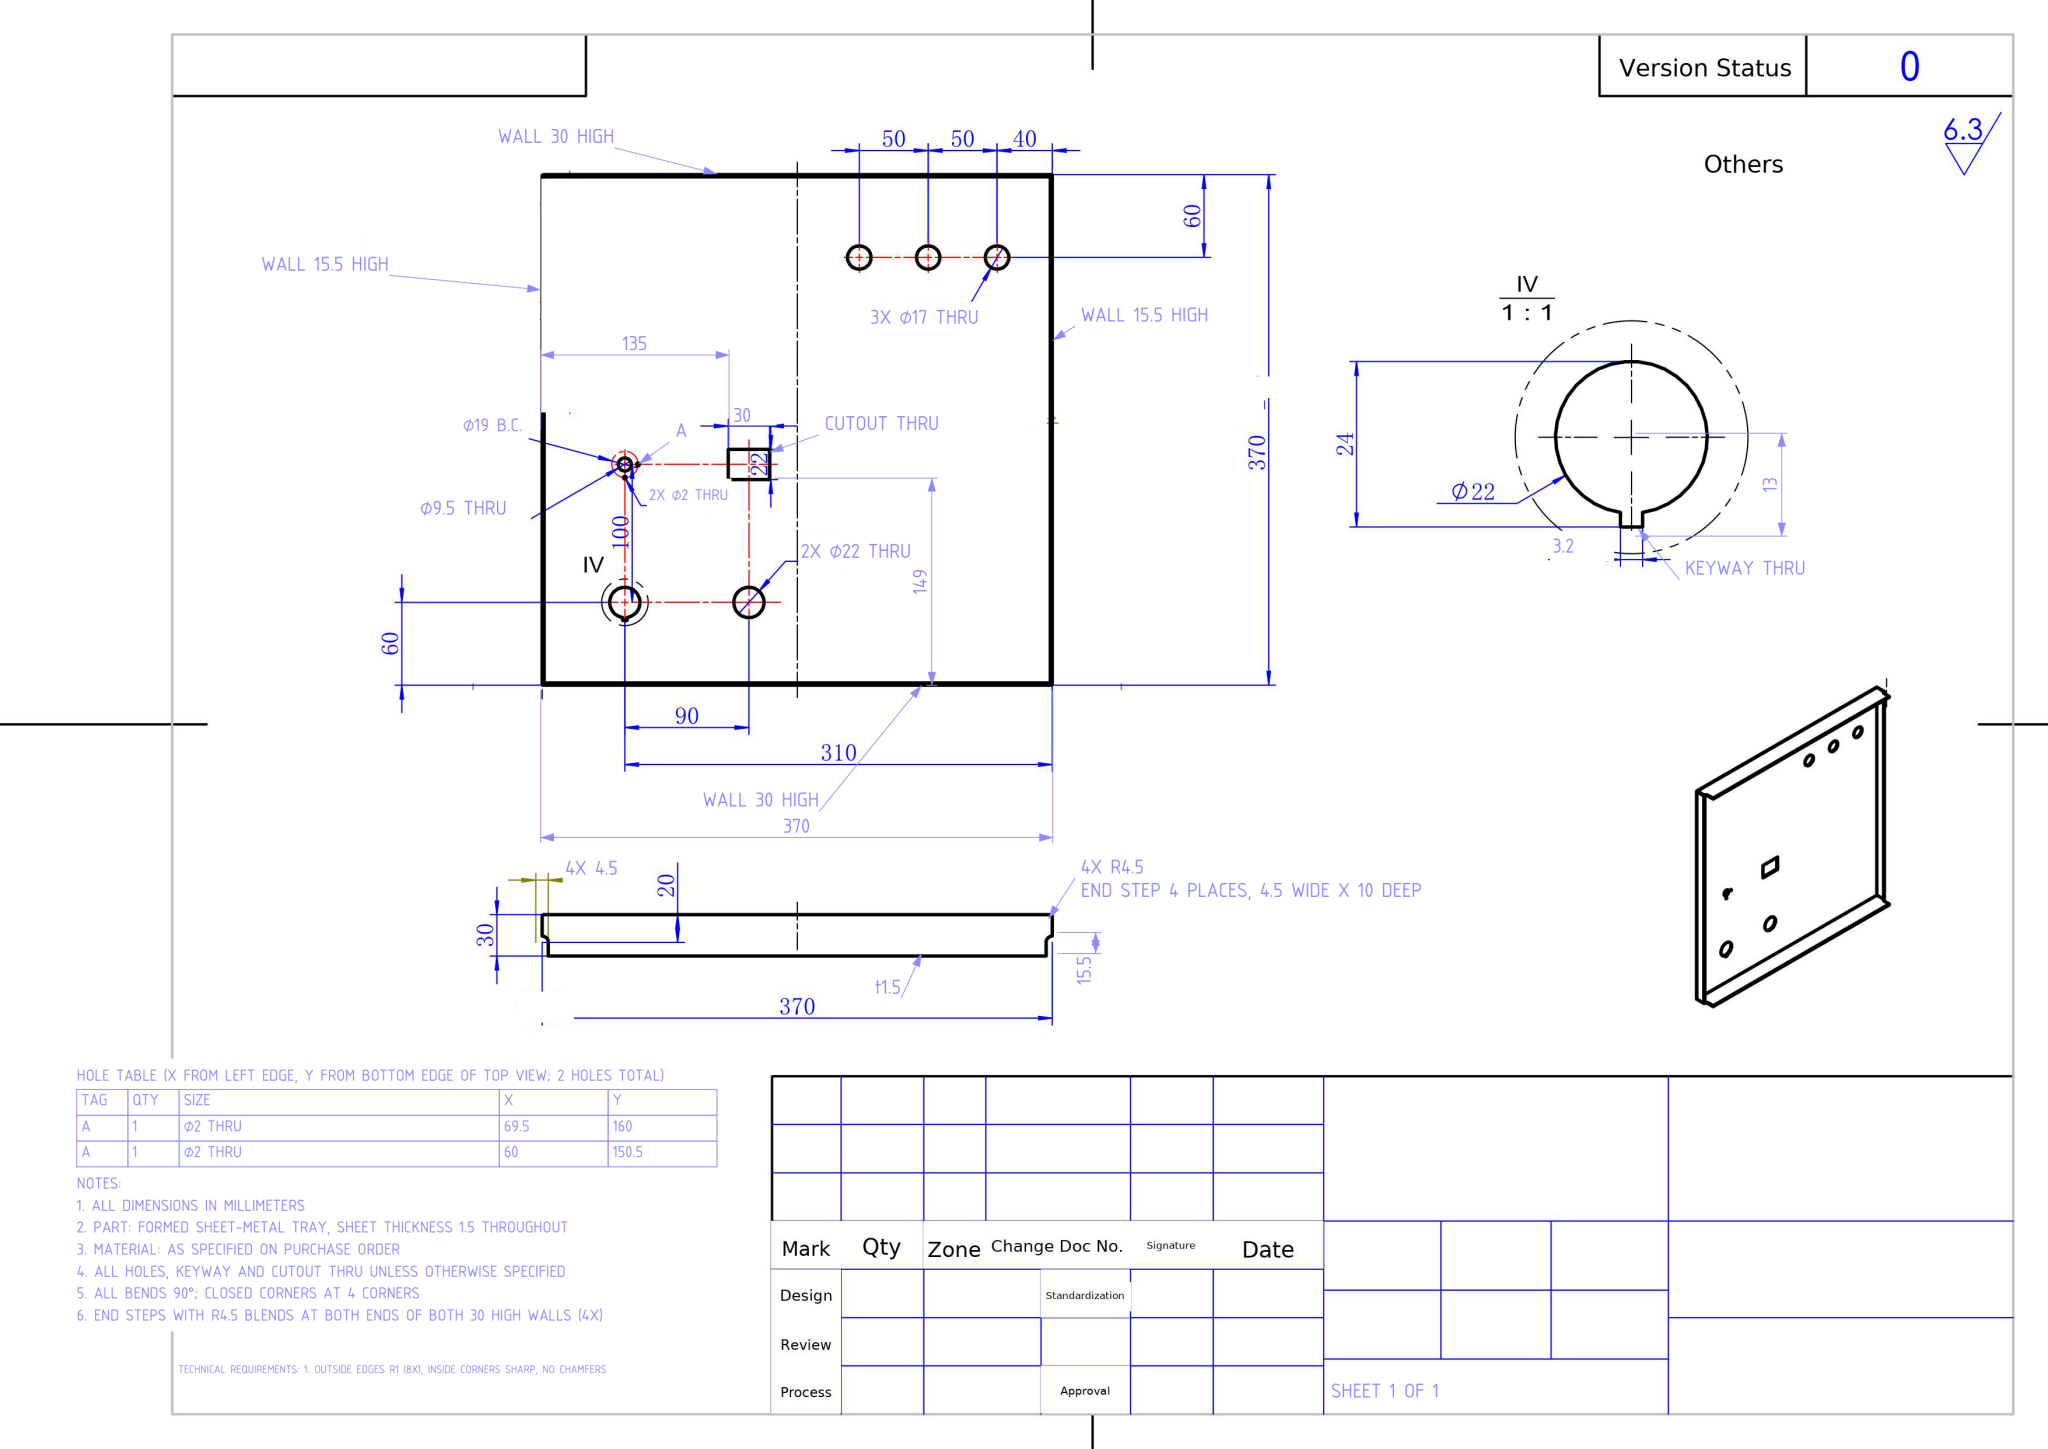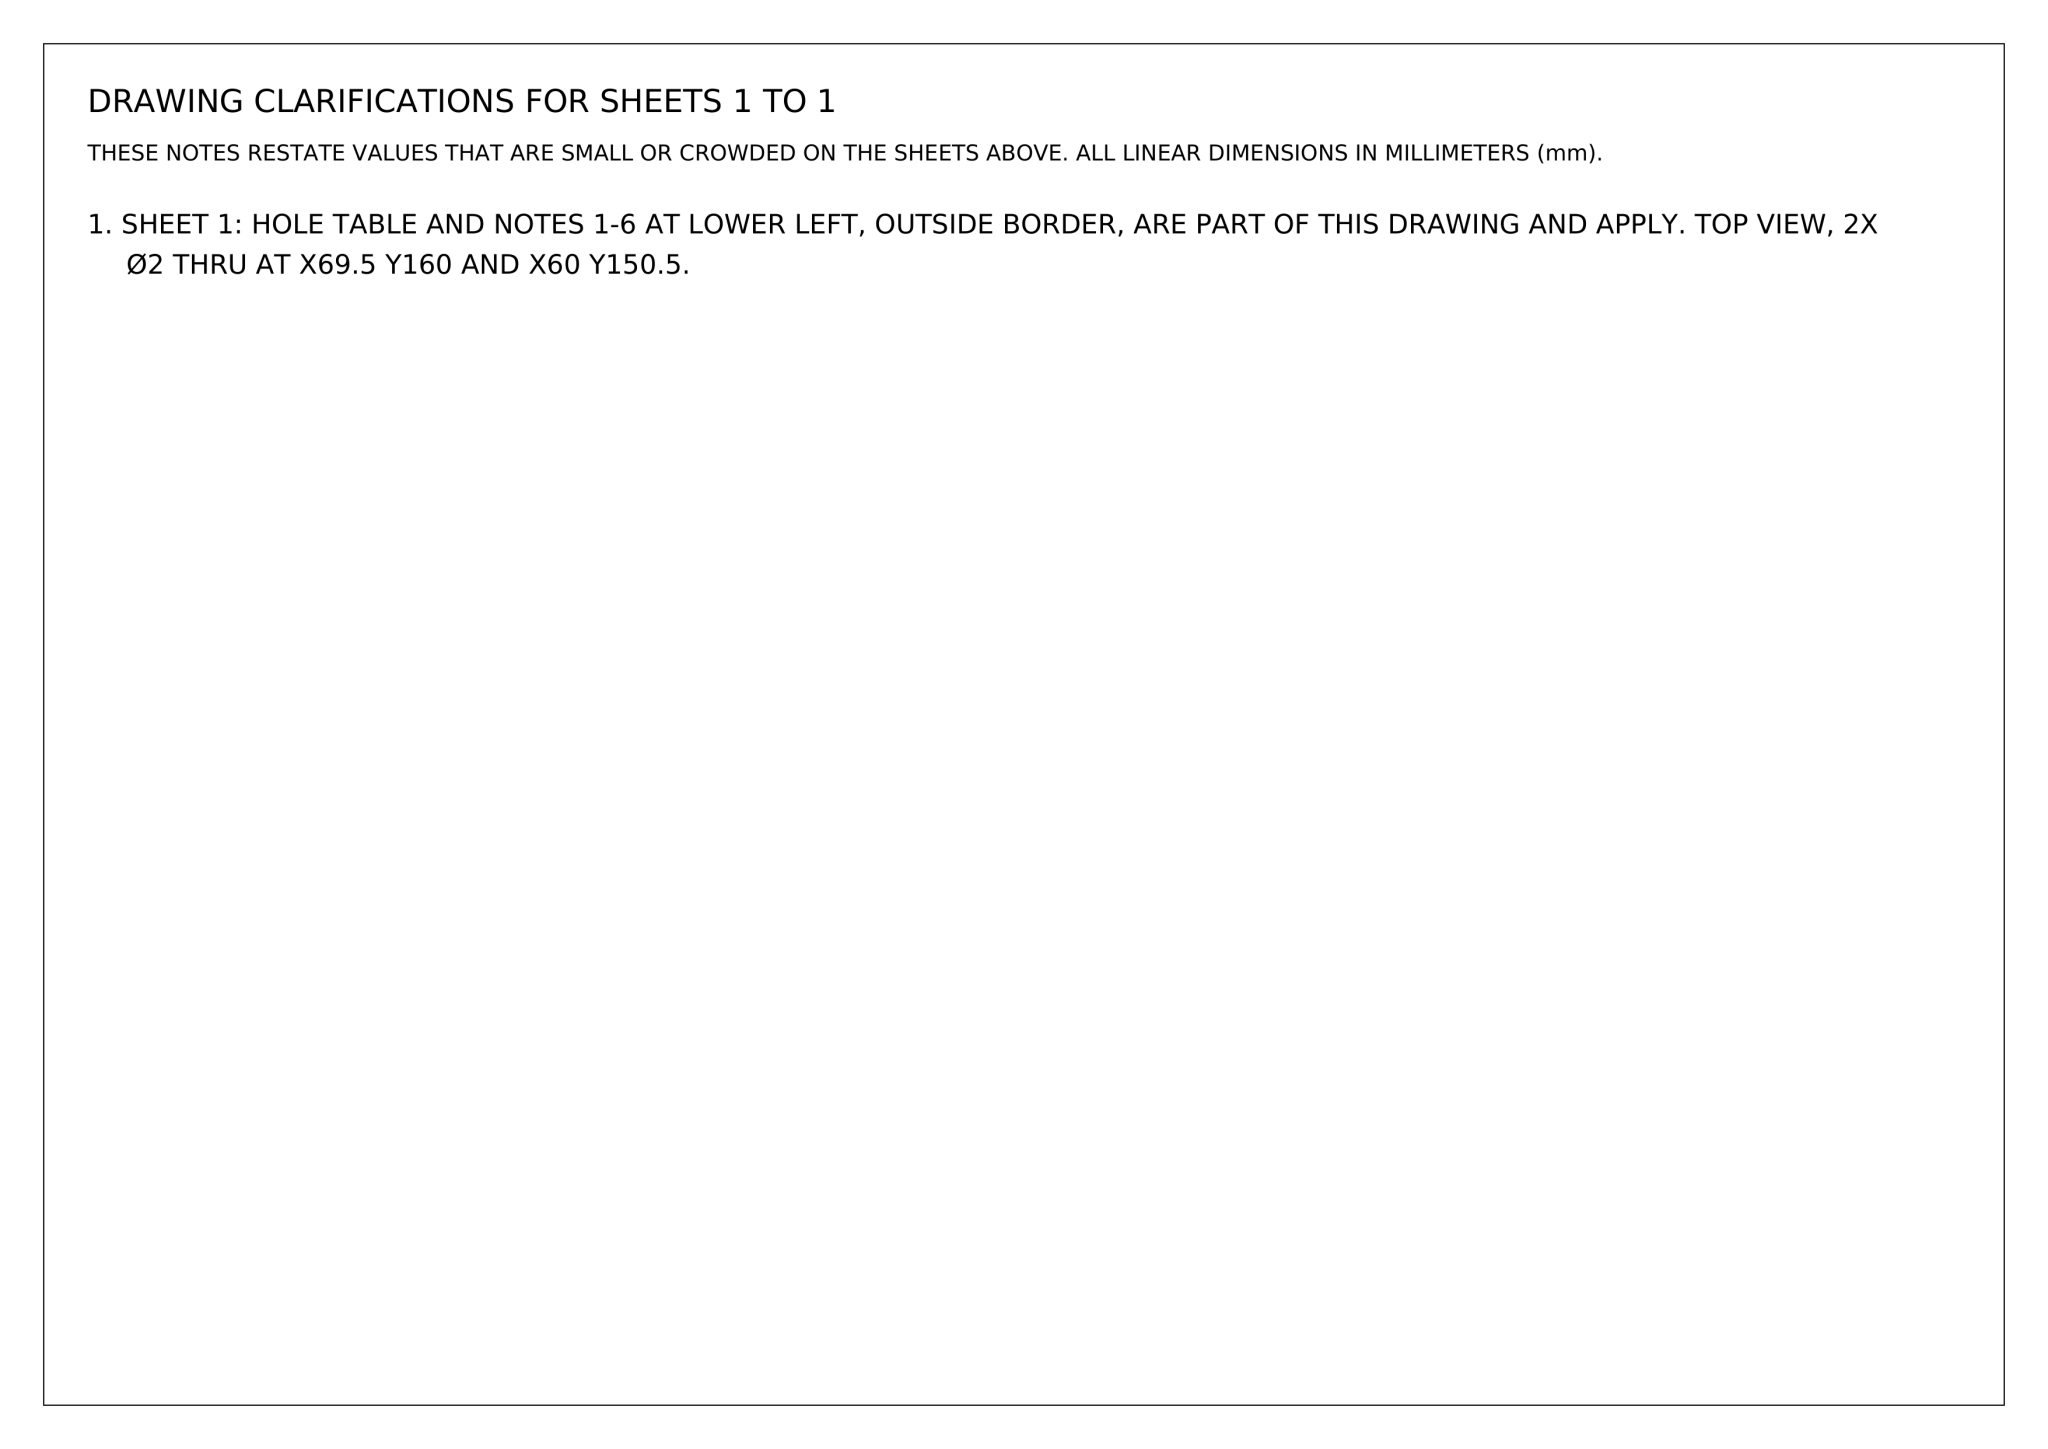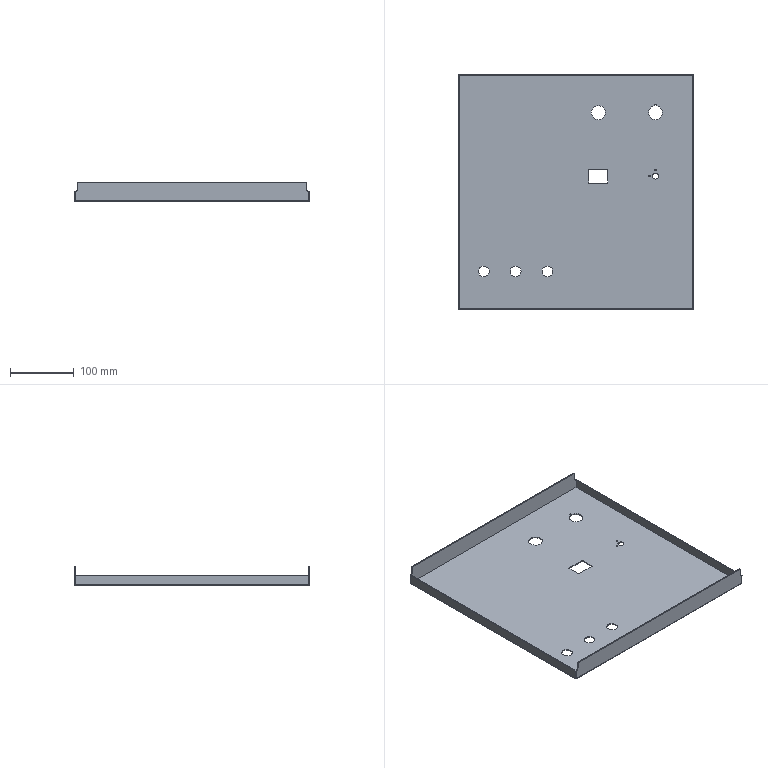Part | NX | mm | 1 solid | 54 faces | box 370 x 370 x 30 mm | volume 248519 mm3 | cylinder 27 | plane 23 | sphere 4 | commonest cylinder face diameters 2 x12 17 x6 22 x5 9.5 x2 9 x2